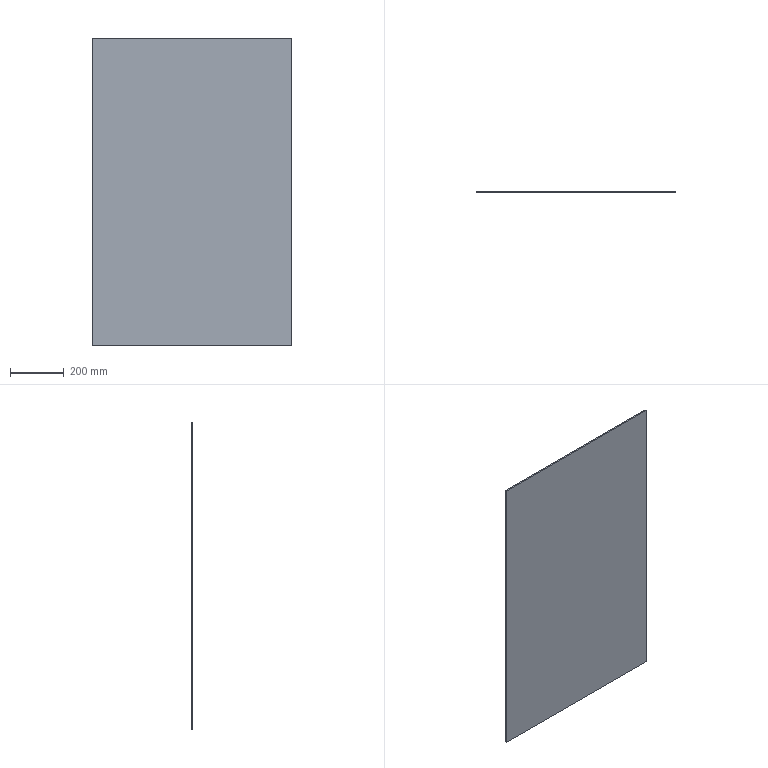Component | SolidWorks | V-GZT-0100-001-1 | 1 solid | 10 faces | box 735 x 5 x 1140 mm | volume 4189393 mm3 | plane 6 | cylinder 4 | commonest cylinder face diameters 10 x4 | material Plexiglas (TM) GS Acrylic Cast Sheet
build123d program:
from build123d import *

# Parameters (mm, degrees)
SKETCH1_W           = 1140
SKETCH1_H           = 735
BOSS_EXTRUDE1_DEPTH = 5
FILLET1_R           = 5


with BuildPart() as part:
    # Sketch1 → Boss-Extrude1 (new body)
    with BuildSketch(Plane.XY):
        Rectangle(SKETCH1_W, SKETCH1_H)
    extrude(amount=BOSS_EXTRUDE1_DEPTH)

    # Fillet1
    fillet1_edges = [part.edges().sort_by_distance(p)[0] for p in [
        (570, -367.5, 2.5),
        (-570, -367.5, 2.5),
        (-570, 367.5, 2.5),
        (570, 367.5, 2.5),
    ]]
    fillet(fillet1_edges, radius=FILLET1_R)


solid = part.part

# Placed as in the assembly
solid = solid.moved(Location((-443.006, 10.587, -1800.428), (90, 0, 90)))
STEP:
#1=CARTESIAN_POINT('',(-3.17,0.4168,-48.442));
#2=VERTEX_POINT('',#1);
#3=CARTESIAN_POINT('',(-31.713,0.4168,-48.442));
#4=VERTEX_POINT('',#3);
#5=CARTESIAN_POINT('',(-31.91,0.4168,-48.442));
#6=DIRECTION('',(-1.,-0.,0.));
#7=VECTOR('',#6,39.37);
#8=LINE('',#5,#7);
#9=EDGE_CURVE('',#2,#4,#8,.T.);
#10=ORIENTED_EDGE('',*,*,#9,.T.);
#11=CARTESIAN_POINT('',(-31.713,0.22,-48.442));
#12=VERTEX_POINT('',#11);
#13=CARTESIAN_POINT('',(-31.713,0.22,-48.442));
#14=DIRECTION('',(0.,-1.,-0.));
#15=VECTOR('',#14,39.37);
#16=LINE('',#13,#15);
#17=EDGE_CURVE('',#4,#12,#16,.T.);
#18=ORIENTED_EDGE('',*,*,#17,.T.);
#19=CARTESIAN_POINT('',(-3.17,0.22,-48.442));
#20=VERTEX_POINT('',#19);
#21=CARTESIAN_POINT('',(-31.91,0.22,-48.442));
#22=DIRECTION('',(-1.,-0.,0.));
#23=VECTOR('',#22,39.37);
#24=LINE('',#21,#23);
#25=EDGE_CURVE('',#20,#12,#24,.T.);
#26=ORIENTED_EDGE('',*,*,#25,.F.);
#27=CARTESIAN_POINT('',(-3.17,0.22,-48.442));
#28=DIRECTION('',(-0.,1.,0.));
#29=VECTOR('',#28,39.37);
#30=LINE('',#27,#29);
#31=EDGE_CURVE('',#20,#2,#30,.T.);
#32=ORIENTED_EDGE('',*,*,#31,.T.);
#33=EDGE_LOOP('',(#10,#18,#26,#32));
#34=FACE_OUTER_BOUND('',#33,.T.);
#35=CARTESIAN_POINT('',(-31.91,0.22,-48.442));
#36=DIRECTION('',(-0.,0.,-1.));
#37=DIRECTION('',(0.,-1.,-0.));
#38=AXIS2_PLACEMENT_3D('',#35,#36,#37);
#39=PLANE('',#38);
#40=ADVANCED_FACE('',(#34),#39,.F.);
#41=CARTESIAN_POINT('',(-31.91,0.22,-48.639));
#42=VERTEX_POINT('',#41);
#43=CARTESIAN_POINT('',(-31.91,0.22,-93.127));
#44=VERTEX_POINT('',#43);
#45=CARTESIAN_POINT('',(-31.91,0.22,-93.324));
#46=DIRECTION('',(-0.,0.,-1.));
#47=VECTOR('',#46,39.37);
#48=LINE('',#45,#47);
#49=EDGE_CURVE('',#42,#44,#48,.T.);
#50=ORIENTED_EDGE('',*,*,#49,.F.);
#51=CARTESIAN_POINT('',(-31.91,0.4168,-48.639));
#52=VERTEX_POINT('',#51);
#53=CARTESIAN_POINT('',(-31.91,0.22,-48.639));
#54=DIRECTION('',(-0.,1.,0.));
#55=VECTOR('',#54,39.37);
#56=LINE('',#53,#55);
#57=EDGE_CURVE('',#42,#52,#56,.T.);
#58=ORIENTED_EDGE('',*,*,#57,.T.);
#59=CARTESIAN_POINT('',(-31.91,0.4168,-93.127));
#60=VERTEX_POINT('',#59);
#61=CARTESIAN_POINT('',(-31.91,0.4168,-93.324));
#62=DIRECTION('',(-0.,0.,-1.));
#63=VECTOR('',#62,39.37);
#64=LINE('',#61,#63);
#65=EDGE_CURVE('',#52,#60,#64,.T.);
#66=ORIENTED_EDGE('',*,*,#65,.T.);
#67=CARTESIAN_POINT('',(-31.91,0.22,-93.127));
#68=DIRECTION('',(0.,-1.,-0.));
#69=VECTOR('',#68,39.37);
#70=LINE('',#67,#69);
#71=EDGE_CURVE('',#60,#44,#70,.T.);
#72=ORIENTED_EDGE('',*,*,#71,.T.);
#73=EDGE_LOOP('',(#50,#58,#66,#72));
#74=FACE_OUTER_BOUND('',#73,.T.);
#75=CARTESIAN_POINT('',(-31.91,0.22,-93.324));
#76=DIRECTION('',(1.,0.,-0.));
#77=DIRECTION('',(-0.,1.,0.));
#78=AXIS2_PLACEMENT_3D('',#75,#76,#77);
#79=PLANE('',#78);
#80=ADVANCED_FACE('',(#74),#79,.F.);
#81=CARTESIAN_POINT('',(-31.713,0.22,-93.324));
#82=VERTEX_POINT('',#81);
#83=CARTESIAN_POINT('',(-3.17,0.22,-93.324));
#84=VERTEX_POINT('',#83);
#85=CARTESIAN_POINT('',(-31.91,0.22,-93.324));
#86=DIRECTION('',(1.,0.,0.));
#87=VECTOR('',#86,39.37);
#88=LINE('',#85,#87);
#89=EDGE_CURVE('',#82,#84,#88,.T.);
#90=ORIENTED_EDGE('',*,*,#89,.F.);
#91=CARTESIAN_POINT('',(-31.713,0.4168,-93.324));
#92=VERTEX_POINT('',#91);
#93=CARTESIAN_POINT('',(-31.713,0.22,-93.324));
#94=DIRECTION('',(-0.,1.,0.));
#95=VECTOR('',#94,39.37);
#96=LINE('',#93,#95);
#97=EDGE_CURVE('',#82,#92,#96,.T.);
#98=ORIENTED_EDGE('',*,*,#97,.T.);
#99=CARTESIAN_POINT('',(-3.17,0.4168,-93.324));
#100=VERTEX_POINT('',#99);
#101=CARTESIAN_POINT('',(-31.91,0.4168,-93.324));
#102=DIRECTION('',(1.,0.,0.));
#103=VECTOR('',#102,39.37);
#104=LINE('',#101,#103);
#105=EDGE_CURVE('',#92,#100,#104,.T.);
#106=ORIENTED_EDGE('',*,*,#105,.T.);
#107=CARTESIAN_POINT('',(-3.17,0.22,-93.324));
#108=DIRECTION('',(0.,-1.,-0.));
#109=VECTOR('',#108,39.37);
#110=LINE('',#107,#109);
#111=EDGE_CURVE('',#100,#84,#110,.T.);
#112=ORIENTED_EDGE('',*,*,#111,.T.);
#113=EDGE_LOOP('',(#90,#98,#106,#112));
#114=FACE_OUTER_BOUND('',#113,.T.);
#115=CARTESIAN_POINT('',(-31.91,0.22,-93.324));
#116=DIRECTION('',(-0.,-0.,1.));
#117=DIRECTION('',(-1.,-0.,-0.));
#118=AXIS2_PLACEMENT_3D('',#115,#116,#117);
#119=PLANE('',#118);
#120=ADVANCED_FACE('',(#114),#119,.F.);
#121=CARTESIAN_POINT('',(-2.973,0.4168,-93.127));
#122=VERTEX_POINT('',#121);
#123=CARTESIAN_POINT('',(-2.973,0.4168,-48.639));
#124=VERTEX_POINT('',#123);
#125=CARTESIAN_POINT('',(-2.973,0.4168,-93.324));
#126=DIRECTION('',(0.,-0.,1.));
#127=VECTOR('',#126,39.37);
#128=LINE('',#125,#127);
#129=EDGE_CURVE('',#122,#124,#128,.T.);
#130=ORIENTED_EDGE('',*,*,#129,.T.);
#131=CARTESIAN_POINT('',(-2.973,0.22,-48.639));
#132=VERTEX_POINT('',#131);
#133=CARTESIAN_POINT('',(-2.973,0.22,-48.639));
#134=DIRECTION('',(0.,-1.,-0.));
#135=VECTOR('',#134,39.37);
#136=LINE('',#133,#135);
#137=EDGE_CURVE('',#124,#132,#136,.T.);
#138=ORIENTED_EDGE('',*,*,#137,.T.);
#139=CARTESIAN_POINT('',(-2.973,0.22,-93.127));
#140=VERTEX_POINT('',#139);
#141=CARTESIAN_POINT('',(-2.973,0.22,-93.324));
#142=DIRECTION('',(0.,-0.,1.));
#143=VECTOR('',#142,39.37);
#144=LINE('',#141,#143);
#145=EDGE_CURVE('',#140,#132,#144,.T.);
#146=ORIENTED_EDGE('',*,*,#145,.F.);
#147=CARTESIAN_POINT('',(-2.973,0.22,-93.127));
#148=DIRECTION('',(-0.,1.,0.));
#149=VECTOR('',#148,39.37);
#150=LINE('',#147,#149);
#151=EDGE_CURVE('',#140,#122,#150,.T.);
#152=ORIENTED_EDGE('',*,*,#151,.T.);
#153=EDGE_LOOP('',(#130,#138,#146,#152));
#154=FACE_OUTER_BOUND('',#153,.T.);
#155=CARTESIAN_POINT('',(-2.973,0.22,-93.324));
#156=DIRECTION('',(-1.,-0.,0.));
#157=DIRECTION('',(-0.,0.,-1.));
#158=AXIS2_PLACEMENT_3D('',#155,#156,#157);
#159=PLANE('',#158);
#160=ADVANCED_FACE('',(#154),#159,.F.);
#161=ORIENTED_EDGE('',*,*,#25,.T.);
#162=CARTESIAN_POINT('',(-31.713,0.22,-48.639));
#163=DIRECTION('',(0.,-1.,-0.));
#164=DIRECTION('',(0.,-0.,1.));
#165=AXIS2_PLACEMENT_3D('',#162,#163,#164);
#166=CIRCLE('',#165,0.1969);
#167=EDGE_CURVE('',#12,#42,#166,.T.);
#168=ORIENTED_EDGE('',*,*,#167,.T.);
#169=ORIENTED_EDGE('',*,*,#49,.T.);
#170=CARTESIAN_POINT('',(-31.713,0.22,-93.127));
#171=DIRECTION('',(0.,-1.,-0.));
#172=DIRECTION('',(0.,-0.,1.));
#173=AXIS2_PLACEMENT_3D('',#170,#171,#172);
#174=CIRCLE('',#173,0.1969);
#175=EDGE_CURVE('',#44,#82,#174,.T.);
#176=ORIENTED_EDGE('',*,*,#175,.T.);
#177=ORIENTED_EDGE('',*,*,#89,.T.);
#178=CARTESIAN_POINT('',(-3.17,0.22,-93.127));
#179=DIRECTION('',(0.,-1.,-0.));
#180=DIRECTION('',(0.,-0.,1.));
#181=AXIS2_PLACEMENT_3D('',#178,#179,#180);
#182=CIRCLE('',#181,0.1969);
#183=EDGE_CURVE('',#84,#140,#182,.T.);
#184=ORIENTED_EDGE('',*,*,#183,.T.);
#185=ORIENTED_EDGE('',*,*,#145,.T.);
#186=CARTESIAN_POINT('',(-3.17,0.22,-48.639));
#187=DIRECTION('',(0.,-1.,-0.));
#188=DIRECTION('',(0.,-0.,1.));
#189=AXIS2_PLACEMENT_3D('',#186,#187,#188);
#190=CIRCLE('',#189,0.1969);
#191=EDGE_CURVE('',#132,#20,#190,.T.);
#192=ORIENTED_EDGE('',*,*,#191,.T.);
#193=EDGE_LOOP('',(#161,#168,#169,#176,#177,#184,#185,#192));
#194=FACE_OUTER_BOUND('',#193,.T.);
#195=CARTESIAN_POINT('',(-17.441,0.22,-70.883));
#196=DIRECTION('',(0.,-1.,-0.));
#197=DIRECTION('',(0.,-0.,1.));
#198=AXIS2_PLACEMENT_3D('',#195,#196,#197);
#199=PLANE('',#198);
#200=ADVANCED_FACE('',(#194),#199,.T.);
#201=ORIENTED_EDGE('',*,*,#65,.F.);
#202=CARTESIAN_POINT('',(-31.713,0.4168,-48.639));
#203=DIRECTION('',(-0.,1.,0.));
#204=DIRECTION('',(0.,0.,1.));
#205=AXIS2_PLACEMENT_3D('',#202,#203,#204);
#206=CIRCLE('',#205,0.1969);
#207=EDGE_CURVE('',#52,#4,#206,.T.);
#208=ORIENTED_EDGE('',*,*,#207,.T.);
#209=ORIENTED_EDGE('',*,*,#9,.F.);
#210=CARTESIAN_POINT('',(-3.17,0.4168,-48.639));
#211=DIRECTION('',(-0.,1.,0.));
#212=DIRECTION('',(0.,0.,1.));
#213=AXIS2_PLACEMENT_3D('',#210,#211,#212);
#214=CIRCLE('',#213,0.1969);
#215=EDGE_CURVE('',#2,#124,#214,.T.);
#216=ORIENTED_EDGE('',*,*,#215,.T.);
#217=ORIENTED_EDGE('',*,*,#129,.F.);
#218=CARTESIAN_POINT('',(-3.17,0.4168,-93.127));
#219=DIRECTION('',(-0.,1.,0.));
#220=DIRECTION('',(0.,0.,1.));
#221=AXIS2_PLACEMENT_3D('',#218,#219,#220);
#222=CIRCLE('',#221,0.1969);
#223=EDGE_CURVE('',#122,#100,#222,.T.);
#224=ORIENTED_EDGE('',*,*,#223,.T.);
#225=ORIENTED_EDGE('',*,*,#105,.F.);
#226=CARTESIAN_POINT('',(-31.713,0.4168,-93.127));
#227=DIRECTION('',(-0.,1.,0.));
#228=DIRECTION('',(0.,0.,1.));
#229=AXIS2_PLACEMENT_3D('',#226,#227,#228);
#230=CIRCLE('',#229,0.1969);
#231=EDGE_CURVE('',#92,#60,#230,.T.);
#232=ORIENTED_EDGE('',*,*,#231,.T.);
#233=EDGE_LOOP('',(#201,#208,#209,#216,#217,#224,#225,#232));
#234=FACE_OUTER_BOUND('',#233,.T.);
#235=CARTESIAN_POINT('',(-17.441,0.4168,-70.883));
#236=DIRECTION('',(0.,-1.,-0.));
#237=DIRECTION('',(0.,-0.,1.));
#238=AXIS2_PLACEMENT_3D('',#235,#236,#237);
#239=PLANE('',#238);
#240=ADVANCED_FACE('',(#234),#239,.F.);
#241=ORIENTED_EDGE('',*,*,#167,.F.);
#242=ORIENTED_EDGE('',*,*,#17,.F.);
#243=ORIENTED_EDGE('',*,*,#207,.F.);
#244=ORIENTED_EDGE('',*,*,#57,.F.);
#245=EDGE_LOOP('',(#241,#242,#243,#244));
#246=FACE_OUTER_BOUND('',#245,.T.);
#247=CARTESIAN_POINT('',(-31.713,0.22,-48.639));
#248=DIRECTION('',(-0.,1.,0.));
#249=DIRECTION('',(0.,0.,-1.));
#250=AXIS2_PLACEMENT_3D('',#247,#248,#249);
#251=CYLINDRICAL_SURFACE('',#250,0.1969);
#252=ADVANCED_FACE('',(#246),#251,.T.);
#253=ORIENTED_EDGE('',*,*,#191,.F.);
#254=ORIENTED_EDGE('',*,*,#137,.F.);
#255=ORIENTED_EDGE('',*,*,#215,.F.);
#256=ORIENTED_EDGE('',*,*,#31,.F.);
#257=EDGE_LOOP('',(#253,#254,#255,#256));
#258=FACE_OUTER_BOUND('',#257,.T.);
#259=CARTESIAN_POINT('',(-3.17,0.22,-48.639));
#260=DIRECTION('',(-0.,1.,0.));
#261=DIRECTION('',(0.,0.,-1.));
#262=AXIS2_PLACEMENT_3D('',#259,#260,#261);
#263=CYLINDRICAL_SURFACE('',#262,0.1969);
#264=ADVANCED_FACE('',(#258),#263,.T.);
#265=ORIENTED_EDGE('',*,*,#175,.F.);
#266=ORIENTED_EDGE('',*,*,#71,.F.);
#267=ORIENTED_EDGE('',*,*,#231,.F.);
#268=ORIENTED_EDGE('',*,*,#97,.F.);
#269=EDGE_LOOP('',(#265,#266,#267,#268));
#270=FACE_OUTER_BOUND('',#269,.T.);
#271=CARTESIAN_POINT('',(-31.713,0.22,-93.127));
#272=DIRECTION('',(-0.,1.,0.));
#273=DIRECTION('',(0.,0.,-1.));
#274=AXIS2_PLACEMENT_3D('',#271,#272,#273);
#275=CYLINDRICAL_SURFACE('',#274,0.1969);
#276=ADVANCED_FACE('',(#270),#275,.T.);
#277=ORIENTED_EDGE('',*,*,#183,.F.);
#278=ORIENTED_EDGE('',*,*,#111,.F.);
#279=ORIENTED_EDGE('',*,*,#223,.F.);
#280=ORIENTED_EDGE('',*,*,#151,.F.);
#281=EDGE_LOOP('',(#277,#278,#279,#280));
#282=FACE_OUTER_BOUND('',#281,.T.);
#283=CARTESIAN_POINT('',(-3.17,0.22,-93.127));
#284=DIRECTION('',(-0.,1.,0.));
#285=DIRECTION('',(0.,0.,-1.));
#286=AXIS2_PLACEMENT_3D('',#283,#284,#285);
#287=CYLINDRICAL_SURFACE('',#286,0.1969);
#288=ADVANCED_FACE('',(#282),#287,.T.);
#289=CLOSED_SHELL('',(#40,#80,#120,#160,#200,#240,#252,#264,#276,#288));
#290=MANIFOLD_SOLID_BREP('',#289);
#291=CARTESIAN_POINT('',(0.,0.,0.));
#292=DIRECTION('',(0.,0.,1.));
#293=DIRECTION('',(1.,0.,0.));
#294=AXIS2_PLACEMENT_3D('',#291,#292,#293);
#295=(LENGTH_UNIT()NAMED_UNIT(*)SI_UNIT($,.METRE.));
#296=LENGTH_MEASURE_WITH_UNIT(LENGTH_MEASURE(0.0254),#295);
#297=DIMENSIONAL_EXPONENTS(1.,0.,0.,0.,0.,0.,0.);
#298=(CONVERSION_BASED_UNIT('',#296)LENGTH_UNIT()NAMED_UNIT(#297));
#299=UNCERTAINTY_MEASURE_WITH_UNIT(LENGTH_MEASURE(0.00001),#298,'','');
#300=(NAMED_UNIT(*)PLANE_ANGLE_UNIT()SI_UNIT($,.RADIAN.));
#301=(NAMED_UNIT(*)SI_UNIT($,.STERADIAN.)SOLID_ANGLE_UNIT());
#302=(GEOMETRIC_REPRESENTATION_CONTEXT(3)GLOBAL_UNCERTAINTY_ASSIGNED_CONTEXT((#299))GLOBAL_UNIT_ASSIGNED_CONTEXT((#298,#300,#301))REPRESENTATION_CONTEXT('',''));
#303=ADVANCED_BREP_SHAPE_REPRESENTATION('',(#290,#294),#302);
#304=COLOUR_RGB('',0.7922,0.8196,0.9333);
#305=FILL_AREA_STYLE_COLOUR('',#304);
#306=FILL_AREA_STYLE('',(#305));
#307=SURFACE_STYLE_FILL_AREA(#306);
#308=SURFACE_SIDE_STYLE('',(#307));
#309=SURFACE_STYLE_USAGE(.BOTH.,#308);
#310=PRESENTATION_STYLE_ASSIGNMENT((#309));
#311=STYLED_ITEM('',(#310),#290);
#312=(LENGTH_UNIT()NAMED_UNIT(*)SI_UNIT($,.METRE.));
#313=LENGTH_MEASURE_WITH_UNIT(LENGTH_MEASURE(0.0254),#312);
#314=DIMENSIONAL_EXPONENTS(1.,0.,0.,0.,0.,0.,0.);
#315=(CONVERSION_BASED_UNIT('',#313)LENGTH_UNIT()NAMED_UNIT(#314));
#316=UNCERTAINTY_MEASURE_WITH_UNIT(LENGTH_MEASURE(0.00001),#315,'','');
#317=(NAMED_UNIT(*)PLANE_ANGLE_UNIT()SI_UNIT($,.RADIAN.));
#318=(NAMED_UNIT(*)SI_UNIT($,.STERADIAN.)SOLID_ANGLE_UNIT());
#319=(GEOMETRIC_REPRESENTATION_CONTEXT(3)GLOBAL_UNCERTAINTY_ASSIGNED_CONTEXT((#316))GLOBAL_UNIT_ASSIGNED_CONTEXT((#315,#317,#318))REPRESENTATION_CONTEXT('',''));
#320=MECHANICAL_DESIGN_GEOMETRIC_PRESENTATION_REPRESENTATION('',(#311),#319);
#321=PRESENTATION_LAYER_ASSIGNMENT('','',(#311));